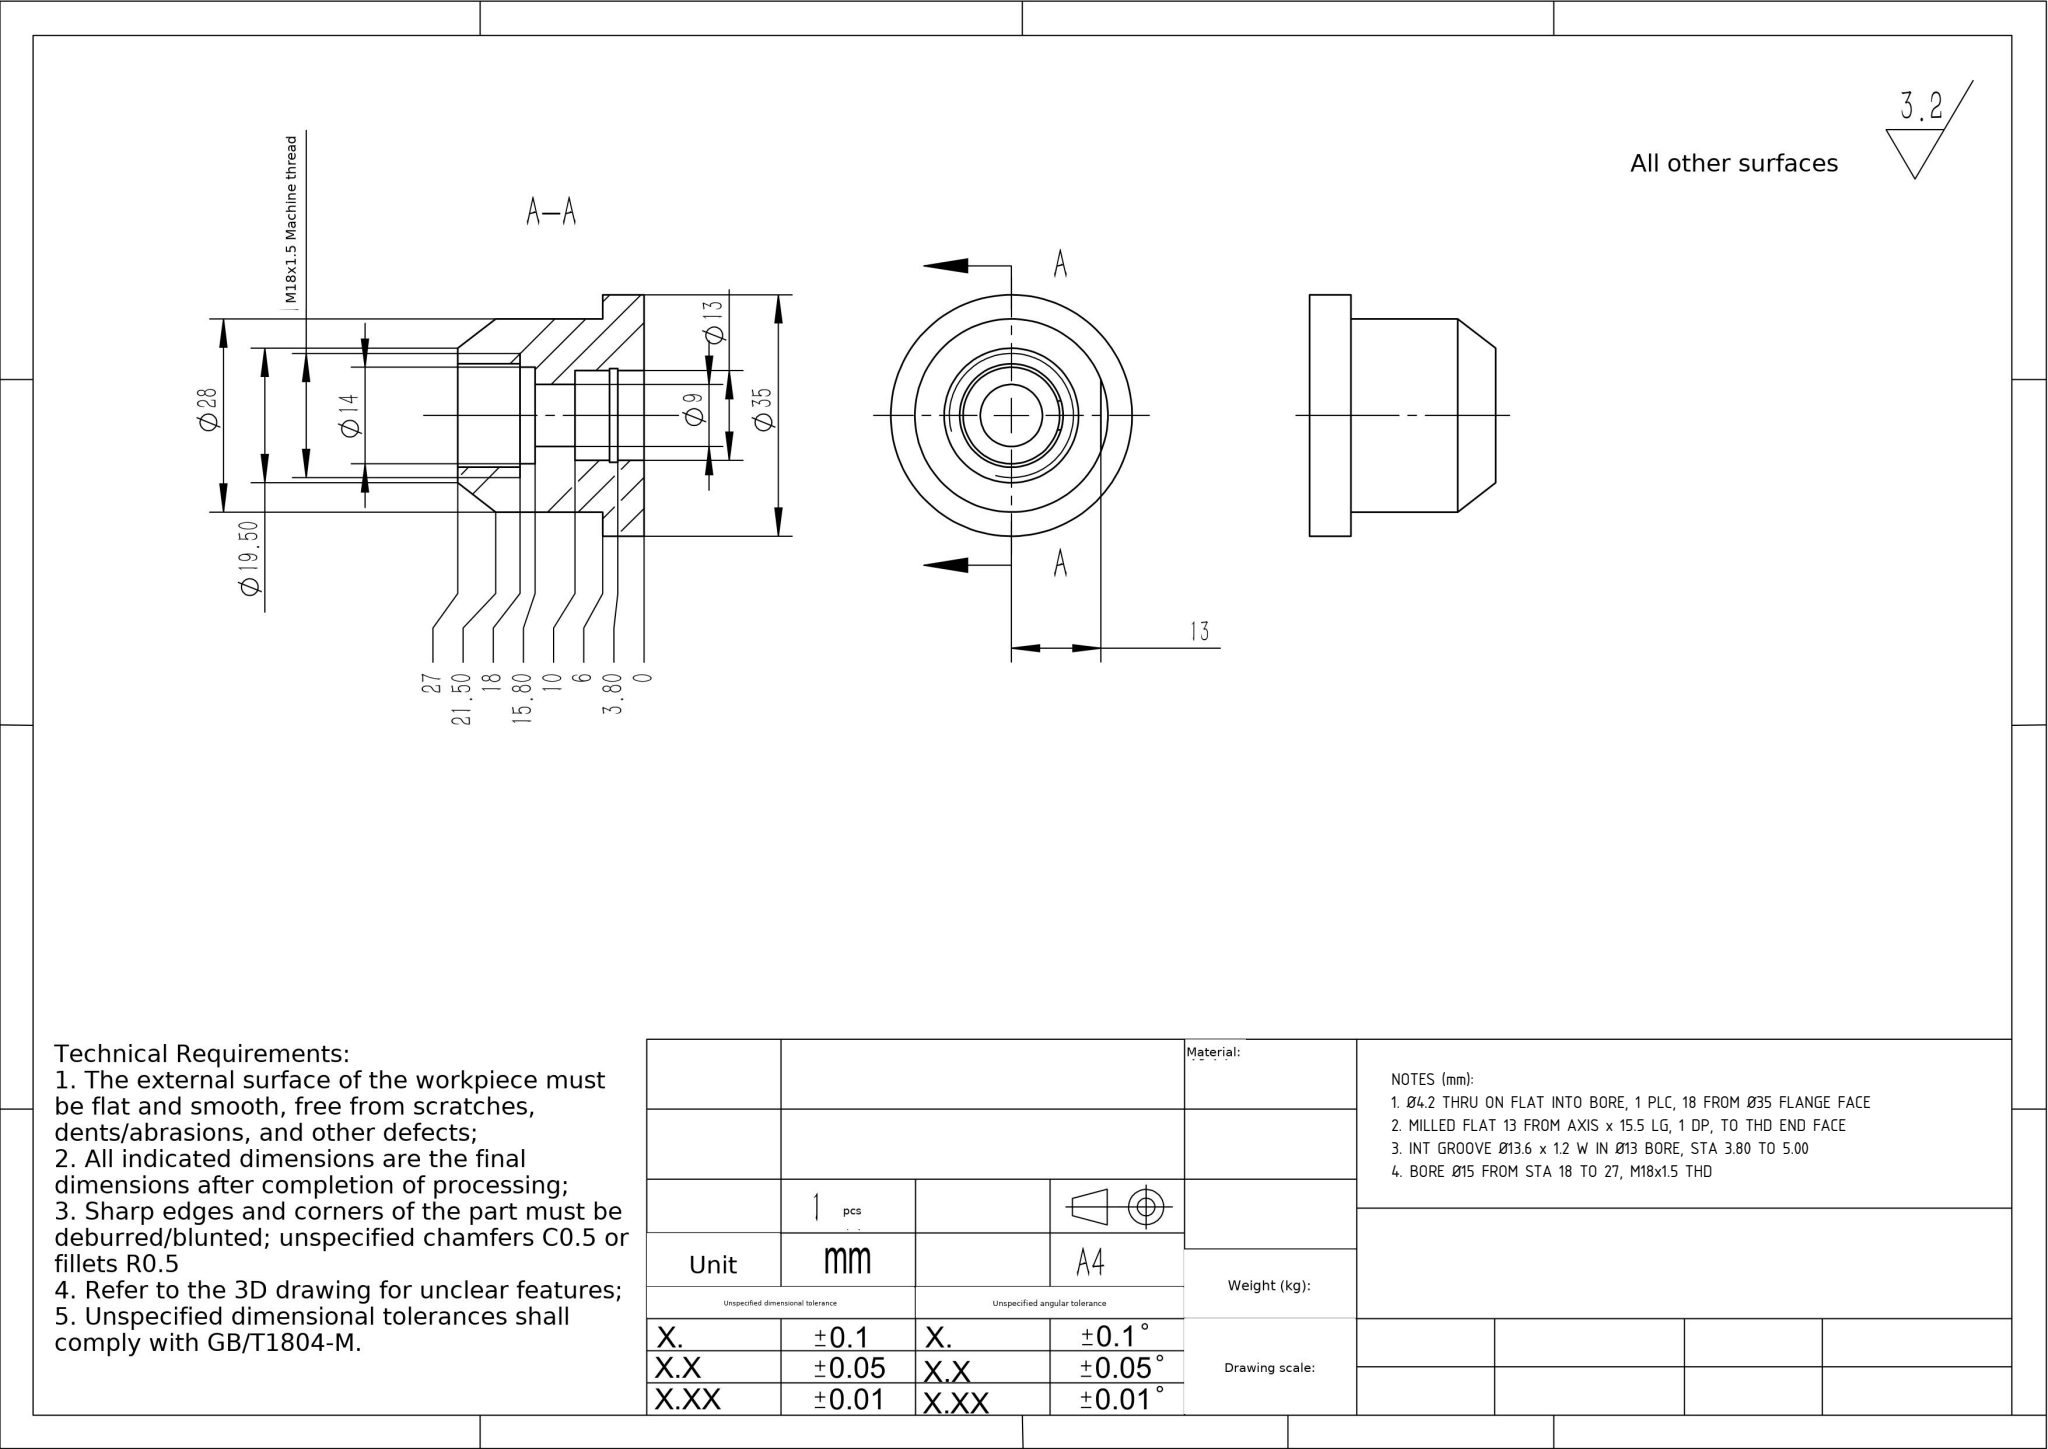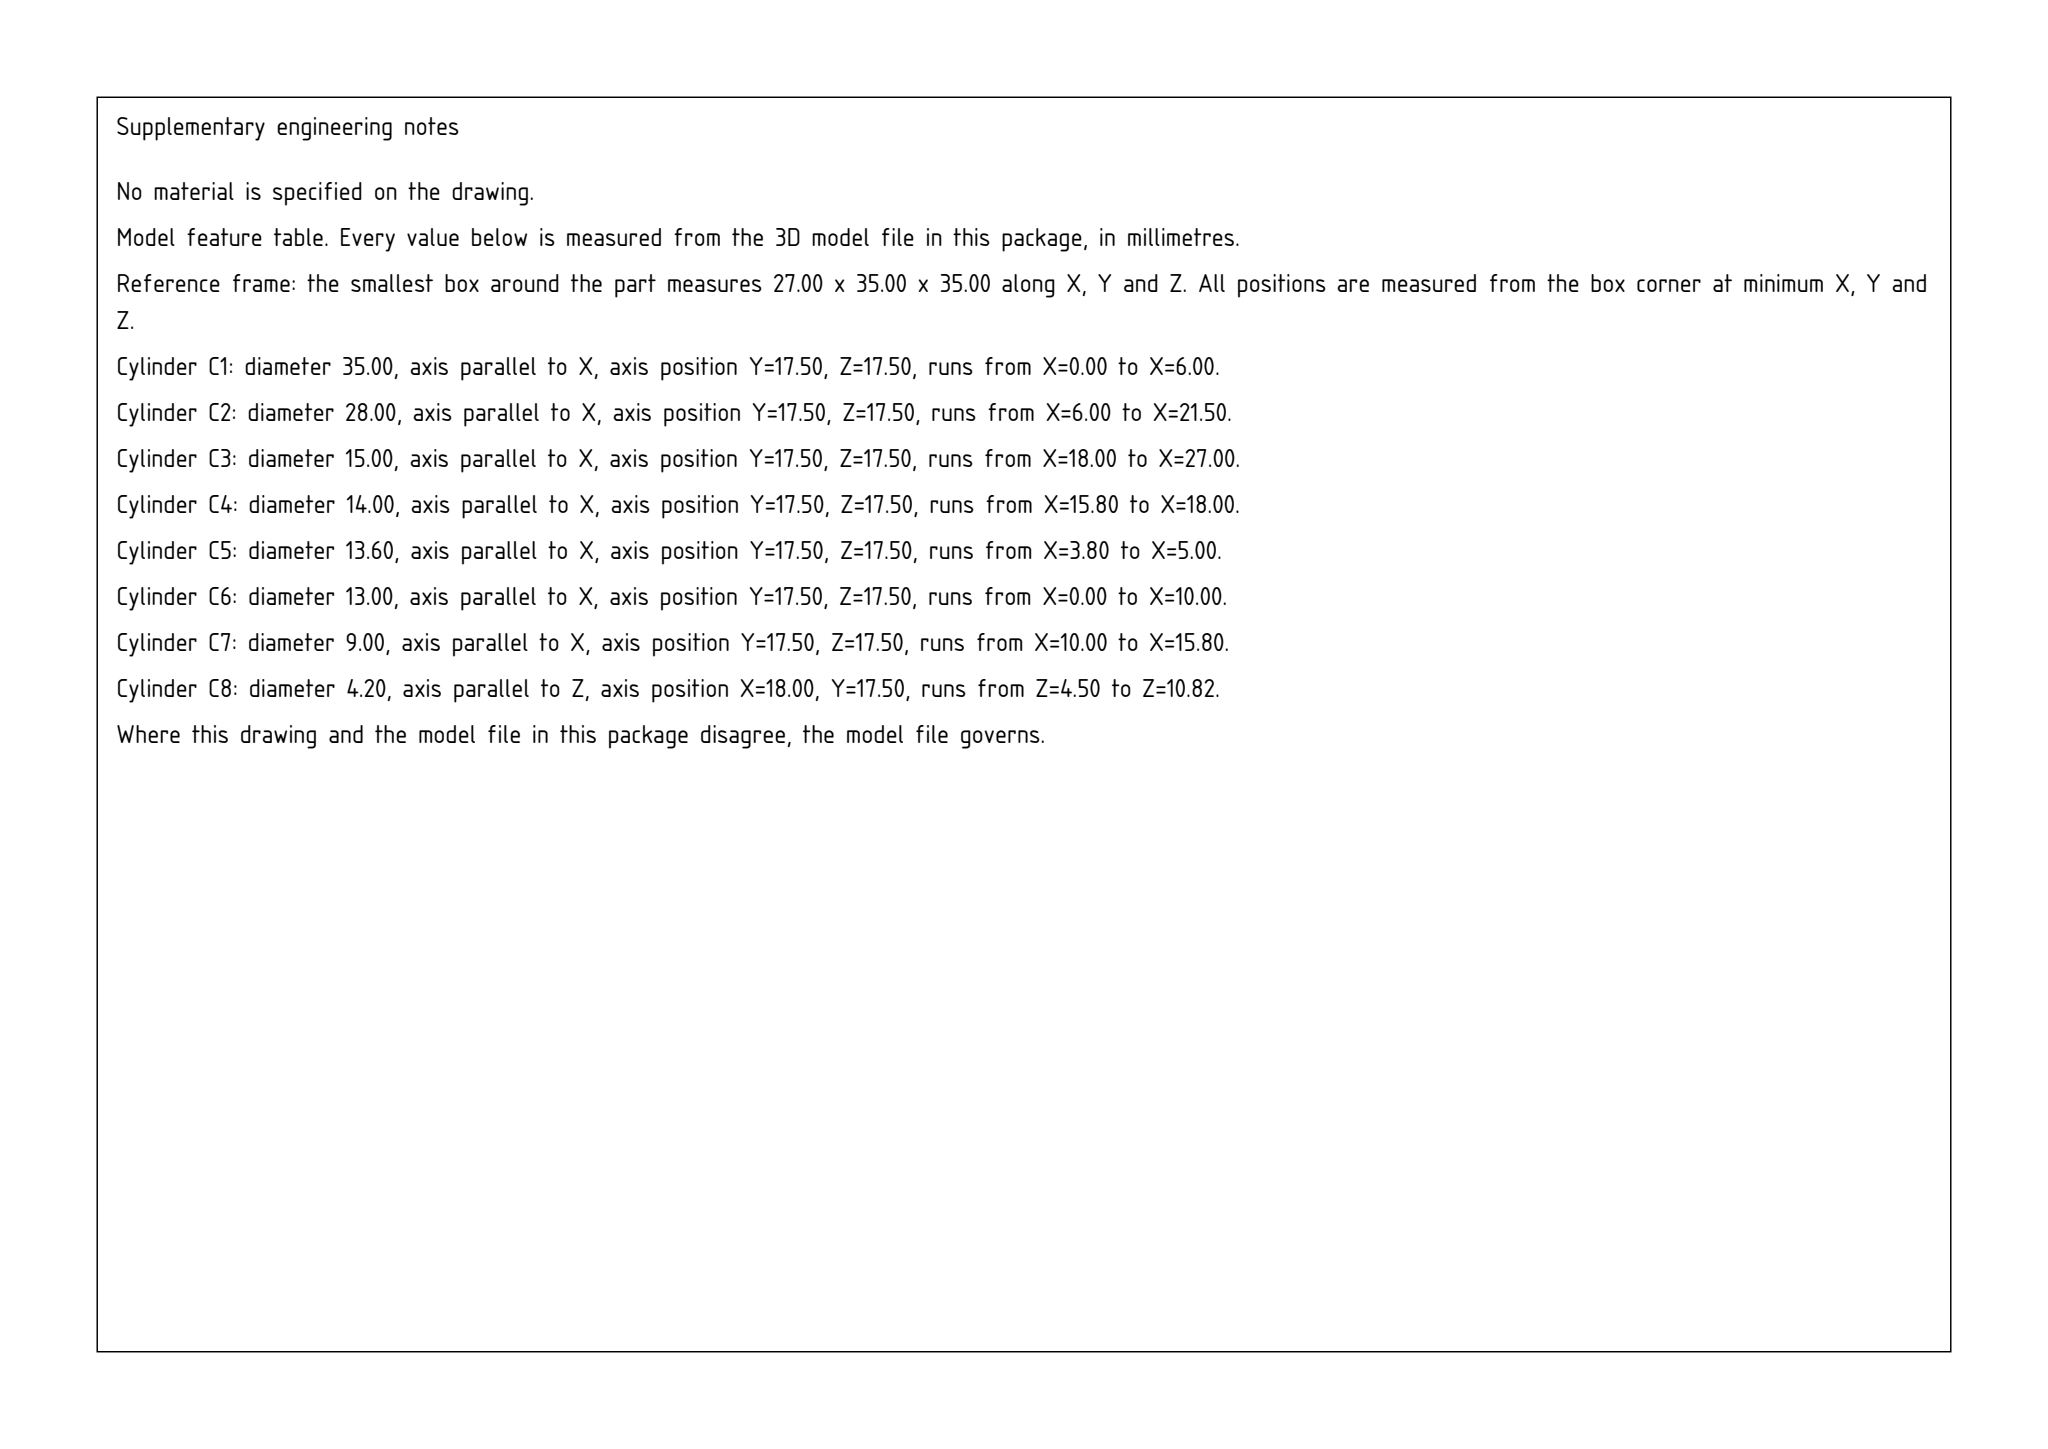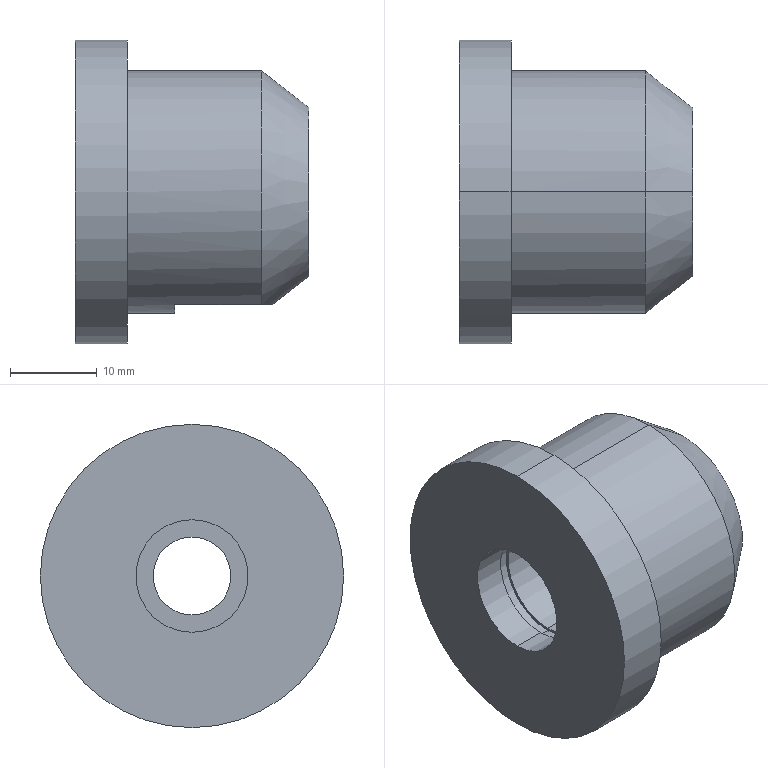Part | SolidWorks | mm | 1 solid | 30 faces | box 27 x 35 x 35 mm | volume 13985 mm3 | cylinder 18 | plane 10 | cone 2 | commonest cylinder face diameters 13 x4 4.2 x2 28 x2 15 x2 14 x2 9 x2 13.6 x2 35 x2
Drawing notes:
Ø4.2 THRU ON FLAT INTO BORE, 1 PLC, 18 FROM Ø35 FLANGE FACE | from the solid: cyl dia 4.2 axis z at x=18.0, y=17.5, len 6.32; starts at flat plane z=4.5, breaks into Ø15/Ø14 bore
MILLED FLAT 13 FROM AXIS x 15.5 LG, 1 DP, TO THD END FACE | from the solid: plane z=4.5 (axis z=17.5 -> 13 offset); Ø28 cyl len 15.5 from x=11.5 (cone end) to x=27 end face; depth 14-13=1
INT GROOVE Ø13.6 x 1.2 W IN Ø13 BORE, STA 3.80 TO 5.00 | from the solid: cyl dia 13.6 len 1.2 between x-planes 3.8 and 5.0, between Ø13 bores (0-3.8 and 5.0-10.0)
BORE Ø15 FROM STA 18 TO 27, M18x1.5 THD | from the solid: cyl dia 15.0 axis x len 9.0 between x-planes 18.0 and 27.0
build123d program:
from build123d import *

# Parameters (mm, degrees)
CUT_EXTRUDE1_DEPTH      = 37.626
CUT_EXTRUDE1_DEPTH_BACK = 37.626
SKETCH2_W               = 16
SKETCH2_H               = 2
M5_TAPPED_HOLE1_D       = 4.2
M5_TAPPED_HOLE1_DEPTH   = 12.4
M5_TAPPED_HOLE1_TIP     = 1.262


with BuildPart() as part:
    # Sketch1 (on Front Plane) → Revolve1 (revolve)
    with BuildSketch(Plane.XY, mode=Mode.PRIVATE) as revolve1_sk:
        Polygon((0, 17.5), (0, 6.5), (3.8, 6.5), (3.8, 6.8), (5, 6.8), (5, 6.5), (10, 6.5), (10, 4.5), (15.8, 4.5), (15.8, 7), (18, 7), (18, 7.5), (27, 7.5), (27, 9.75), (21.5, 14), (6, 14), (6, 17.5), align=None)
    revolve(revolve1_sk.sketch.rotate(Axis((0, 0, 0), (1, 0, 0)), 90), axis=Axis((0, 0, 0), (1, 0, 0)))

    # Sketch2 → Cut-Extrude1 (cut, two sides: drawn at the far end of the back side and taken through both)
    with BuildSketch(Plane(origin=(0, 0, 0), x_dir=(1, 0, 0), z_dir=(0, 1, 0)).offset(-CUT_EXTRUDE1_DEPTH_BACK)):
        with Locations((19.5, 14)):
            Rectangle(SKETCH2_W, SKETCH2_H)
    extrude(amount=CUT_EXTRUDE1_DEPTH + CUT_EXTRUDE1_DEPTH_BACK, mode=Mode.SUBTRACT)

    # M5 Tapped Hole1
    with Locations(Plane(origin=(18, 0, -13), x_dir=(-1, 0, 0), z_dir=(0, 0, -1))):
        with Locations((0, 0)):
            Hole(M5_TAPPED_HOLE1_D / 2, depth=M5_TAPPED_HOLE1_DEPTH)
            with Locations((0, 0, -(M5_TAPPED_HOLE1_DEPTH + M5_TAPPED_HOLE1_TIP / 2))):  # 118° drill point
                Cone(0, M5_TAPPED_HOLE1_D / 2, M5_TAPPED_HOLE1_TIP, mode=Mode.SUBTRACT)


solid = part.part